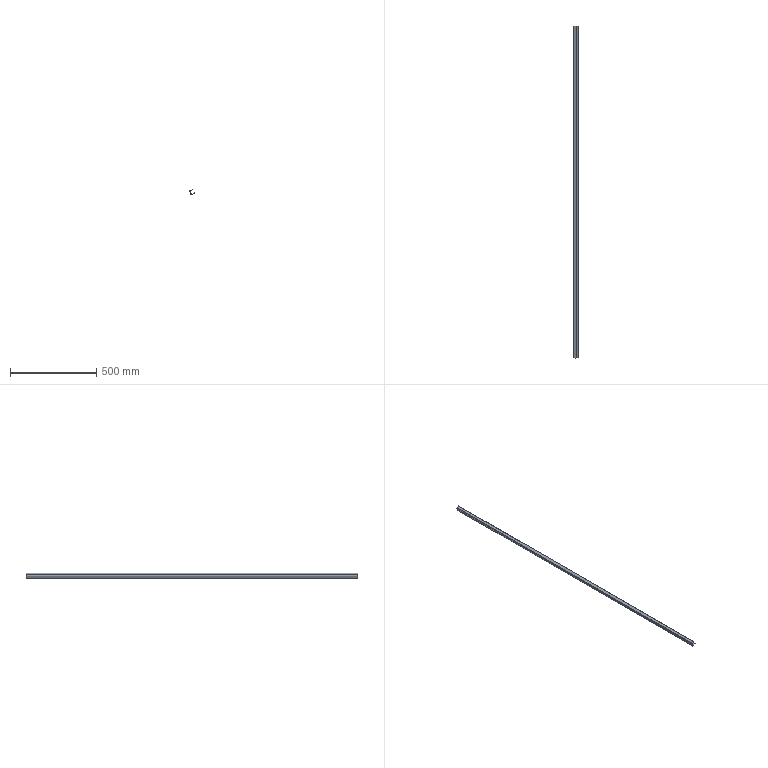Component | SolidWorks | FrontDoorAssembly-1_DoorLeftAndRightReinforcementBar-2 | 1 solid | 22 faces | box 27.81 x 1920 x 29.64 mm | volume 219407 mm3 | plane 18 | cylinder 4 | commonest cylinder face diameters 11 x2 7 x2 | material Malleable Cast Iron
STEP:
#1=COLOUR_RGB('',0.7922,0.8196,0.9333);
#2=FILL_AREA_STYLE_COLOUR('',#1);
#3=FILL_AREA_STYLE('',(#2));
#4=SURFACE_STYLE_FILL_AREA(#3);
#5=SURFACE_SIDE_STYLE('',(#4));
#6=SURFACE_STYLE_USAGE(.BOTH.,#5);
#7=PRESENTATION_STYLE_ASSIGNMENT((#6));
#8=CARTESIAN_POINT('',(-2.645,74.27,40.544));
#9=VERTEX_POINT('',#8);
#10=CARTESIAN_POINT('',(-2.577,74.27,40.583));
#11=VERTEX_POINT('',#10);
#12=CARTESIAN_POINT('',(-2.645,74.27,40.544));
#13=DIRECTION('',(0.866,0.,0.5));
#14=VECTOR('',#13,39.37);
#15=LINE('',#12,#14);
#16=EDGE_CURVE('',#9,#11,#15,.T.);
#17=ORIENTED_EDGE('',*,*,#16,.F.);
#18=CARTESIAN_POINT('',(-2.566,74.27,40.84));
#19=VERTEX_POINT('',#18);
#20=CARTESIAN_POINT('',(-2.458,74.27,40.652));
#21=DIRECTION('',(0.,-1.,-0.));
#22=DIRECTION('',(0.866,0.,0.5));
#23=AXIS2_PLACEMENT_3D('',#20,#21,#22);
#24=CIRCLE('',#23,0.2165);
#25=EDGE_CURVE('',#19,#9,#24,.T.);
#26=ORIENTED_EDGE('',*,*,#25,.F.);
#27=CARTESIAN_POINT('',(-2.527,74.27,40.771));
#28=VERTEX_POINT('',#27);
#29=CARTESIAN_POINT('',(-2.527,74.27,40.771));
#30=DIRECTION('',(-0.5,-0.,0.866));
#31=VECTOR('',#30,39.37);
#32=LINE('',#29,#31);
#33=EDGE_CURVE('',#28,#19,#32,.T.);
#34=ORIENTED_EDGE('',*,*,#33,.F.);
#35=CARTESIAN_POINT('',(-2.458,74.27,40.652));
#36=DIRECTION('',(0.,-1.,-0.));
#37=DIRECTION('',(0.5,0.,-0.866));
#38=AXIS2_PLACEMENT_3D('',#35,#36,#37);
#39=CIRCLE('',#38,0.1378);
#40=EDGE_CURVE('',#28,#11,#39,.T.);
#41=ORIENTED_EDGE('',*,*,#40,.T.);
#42=EDGE_LOOP('',(#17,#26,#34,#41));
#43=FACE_OUTER_BOUND('',#42,.T.);
#44=CARTESIAN_POINT('',(-2.645,74.27,40.544));
#45=DIRECTION('',(-0.,1.,0.));
#46=DIRECTION('',(0.866,0.,0.5));
#47=AXIS2_PLACEMENT_3D('',#44,#45,#46);
#48=PLANE('',#47);
#49=ADVANCED_FACE('',(#43),#48,.T.);
#50=CARTESIAN_POINT('',(-2.37,74.27,40.067));
#51=VERTEX_POINT('',#50);
#52=CARTESIAN_POINT('',(-2.754,74.27,40.731));
#53=DIRECTION('',(0.5,0.,-0.866));
#54=VECTOR('',#53,39.37);
#55=LINE('',#52,#54);
#56=EDGE_CURVE('',#9,#51,#55,.T.);
#57=ORIENTED_EDGE('',*,*,#56,.F.);
#58=ORIENTED_EDGE('',*,*,#16,.T.);
#59=CARTESIAN_POINT('',(-2.302,74.27,40.106));
#60=VERTEX_POINT('',#59);
#61=CARTESIAN_POINT('',(-2.686,74.27,40.771));
#62=DIRECTION('',(0.5,0.,-0.866));
#63=VECTOR('',#62,39.37);
#64=LINE('',#61,#63);
#65=EDGE_CURVE('',#11,#60,#64,.T.);
#66=ORIENTED_EDGE('',*,*,#65,.T.);
#67=CARTESIAN_POINT('',(-2.302,74.27,40.106));
#68=DIRECTION('',(-0.866,-0.,-0.5));
#69=VECTOR('',#68,39.37);
#70=LINE('',#67,#69);
#71=EDGE_CURVE('',#60,#51,#70,.T.);
#72=ORIENTED_EDGE('',*,*,#71,.T.);
#73=EDGE_LOOP('',(#57,#58,#66,#72));
#74=FACE_OUTER_BOUND('',#73,.T.);
#75=CARTESIAN_POINT('',(-2.527,74.27,40.771));
#76=DIRECTION('',(-0.,1.,0.));
#77=DIRECTION('',(0.866,0.,0.5));
#78=AXIS2_PLACEMENT_3D('',#75,#76,#77);
#79=PLANE('',#78);
#80=ADVANCED_FACE('',(#74),#79,.T.);
#81=CARTESIAN_POINT('',(-2.566,-1.32,40.84));
#82=VERTEX_POINT('',#81);
#83=CARTESIAN_POINT('',(-2.527,-1.32,40.771));
#84=VERTEX_POINT('',#83);
#85=CARTESIAN_POINT('',(-2.566,-1.32,40.84));
#86=DIRECTION('',(0.5,0.,-0.866));
#87=VECTOR('',#86,39.37);
#88=LINE('',#85,#87);
#89=EDGE_CURVE('',#82,#84,#88,.T.);
#90=ORIENTED_EDGE('',*,*,#89,.F.);
#91=CARTESIAN_POINT('',(-2.645,-1.32,40.544));
#92=VERTEX_POINT('',#91);
#93=CARTESIAN_POINT('',(-2.458,-1.32,40.652));
#94=DIRECTION('',(0.,-1.,-0.));
#95=DIRECTION('',(0.866,0.,0.5));
#96=AXIS2_PLACEMENT_3D('',#93,#94,#95);
#97=CIRCLE('',#96,0.2165);
#98=EDGE_CURVE('',#82,#92,#97,.T.);
#99=ORIENTED_EDGE('',*,*,#98,.T.);
#100=CARTESIAN_POINT('',(-2.577,-1.32,40.583));
#101=VERTEX_POINT('',#100);
#102=CARTESIAN_POINT('',(-2.577,-1.32,40.583));
#103=DIRECTION('',(-0.866,-0.,-0.5));
#104=VECTOR('',#103,39.37);
#105=LINE('',#102,#104);
#106=EDGE_CURVE('',#101,#92,#105,.T.);
#107=ORIENTED_EDGE('',*,*,#106,.F.);
#108=CARTESIAN_POINT('',(-2.458,-1.32,40.652));
#109=DIRECTION('',(0.,-1.,-0.));
#110=DIRECTION('',(0.5,0.,-0.866));
#111=AXIS2_PLACEMENT_3D('',#108,#109,#110);
#112=CIRCLE('',#111,0.1378);
#113=EDGE_CURVE('',#84,#101,#112,.T.);
#114=ORIENTED_EDGE('',*,*,#113,.F.);
#115=EDGE_LOOP('',(#90,#99,#107,#114));
#116=FACE_OUTER_BOUND('',#115,.T.);
#117=CARTESIAN_POINT('',(-2.566,-1.32,40.84));
#118=DIRECTION('',(0.,-1.,-0.));
#119=DIRECTION('',(-0.866,-0.,-0.5));
#120=AXIS2_PLACEMENT_3D('',#117,#118,#119);
#121=PLANE('',#120);
#122=ADVANCED_FACE('',(#116),#121,.T.);
#123=CARTESIAN_POINT('',(-2.072,-1.32,41.125));
#124=VERTEX_POINT('',#123);
#125=CARTESIAN_POINT('',(-2.072,-1.32,41.125));
#126=DIRECTION('',(-0.866,-0.,-0.5));
#127=VECTOR('',#126,39.37);
#128=LINE('',#125,#127);
#129=EDGE_CURVE('',#124,#82,#128,.T.);
#130=ORIENTED_EDGE('',*,*,#129,.T.);
#131=ORIENTED_EDGE('',*,*,#89,.T.);
#132=CARTESIAN_POINT('',(-2.032,-1.32,41.057));
#133=VERTEX_POINT('',#132);
#134=CARTESIAN_POINT('',(-2.032,-1.32,41.057));
#135=DIRECTION('',(-0.866,-0.,-0.5));
#136=VECTOR('',#135,39.37);
#137=LINE('',#134,#136);
#138=EDGE_CURVE('',#133,#84,#137,.T.);
#139=ORIENTED_EDGE('',*,*,#138,.F.);
#140=CARTESIAN_POINT('',(-2.032,-1.32,41.057));
#141=DIRECTION('',(-0.5,-0.,0.866));
#142=VECTOR('',#141,39.37);
#143=LINE('',#140,#142);
#144=EDGE_CURVE('',#133,#124,#143,.T.);
#145=ORIENTED_EDGE('',*,*,#144,.T.);
#146=EDGE_LOOP('',(#130,#131,#139,#145));
#147=FACE_OUTER_BOUND('',#146,.T.);
#148=CARTESIAN_POINT('',(-2.577,-1.32,40.583));
#149=DIRECTION('',(0.,-1.,-0.));
#150=DIRECTION('',(-0.866,-0.,-0.5));
#151=AXIS2_PLACEMENT_3D('',#148,#149,#150);
#152=PLANE('',#151);
#153=ADVANCED_FACE('',(#147),#152,.T.);
#154=CARTESIAN_POINT('',(-2.074,74.27,39.987));
#155=VERTEX_POINT('',#154);
#156=CARTESIAN_POINT('',(-2.113,74.27,40.055));
#157=VERTEX_POINT('',#156);
#158=CARTESIAN_POINT('',(-2.074,74.27,39.987));
#159=DIRECTION('',(-0.5,-0.,0.866));
#160=VECTOR('',#159,39.37);
#161=LINE('',#158,#160);
#162=EDGE_CURVE('',#155,#157,#161,.T.);
#163=ORIENTED_EDGE('',*,*,#162,.F.);
#164=CARTESIAN_POINT('',(-2.182,74.27,40.175));
#165=DIRECTION('',(0.,-1.,-0.));
#166=DIRECTION('',(0.866,0.,0.5));
#167=AXIS2_PLACEMENT_3D('',#164,#165,#166);
#168=CIRCLE('',#167,0.2165);
#169=EDGE_CURVE('',#51,#155,#168,.T.);
#170=ORIENTED_EDGE('',*,*,#169,.F.);
#171=ORIENTED_EDGE('',*,*,#71,.F.);
#172=CARTESIAN_POINT('',(-2.182,74.27,40.175));
#173=DIRECTION('',(0.,-1.,-0.));
#174=DIRECTION('',(0.5,0.,-0.866));
#175=AXIS2_PLACEMENT_3D('',#172,#173,#174);
#176=CIRCLE('',#175,0.1378);
#177=EDGE_CURVE('',#60,#157,#176,.T.);
#178=ORIENTED_EDGE('',*,*,#177,.T.);
#179=EDGE_LOOP('',(#163,#170,#171,#178));
#180=FACE_OUTER_BOUND('',#179,.T.);
#181=CARTESIAN_POINT('',(-2.074,74.27,39.987));
#182=DIRECTION('',(-0.,1.,0.));
#183=DIRECTION('',(0.866,0.,0.5));
#184=AXIS2_PLACEMENT_3D('',#181,#182,#183);
#185=PLANE('',#184);
#186=ADVANCED_FACE('',(#180),#185,.T.);
#187=CARTESIAN_POINT('',(-1.58,74.27,40.273));
#188=VERTEX_POINT('',#187);
#189=CARTESIAN_POINT('',(-2.262,74.27,39.879));
#190=DIRECTION('',(0.866,0.,0.5));
#191=VECTOR('',#190,39.37);
#192=LINE('',#189,#191);
#193=EDGE_CURVE('',#155,#188,#192,.T.);
#194=ORIENTED_EDGE('',*,*,#193,.F.);
#195=ORIENTED_EDGE('',*,*,#162,.T.);
#196=CARTESIAN_POINT('',(-1.619,74.27,40.341));
#197=VERTEX_POINT('',#196);
#198=CARTESIAN_POINT('',(-2.301,74.27,39.947));
#199=DIRECTION('',(0.866,0.,0.5));
#200=VECTOR('',#199,39.37);
#201=LINE('',#198,#200);
#202=EDGE_CURVE('',#157,#197,#201,.T.);
#203=ORIENTED_EDGE('',*,*,#202,.T.);
#204=CARTESIAN_POINT('',(-1.58,74.27,40.273));
#205=DIRECTION('',(-0.5,-0.,0.866));
#206=VECTOR('',#205,39.37);
#207=LINE('',#204,#206);
#208=EDGE_CURVE('',#188,#197,#207,.T.);
#209=ORIENTED_EDGE('',*,*,#208,.F.);
#210=EDGE_LOOP('',(#194,#195,#203,#209));
#211=FACE_OUTER_BOUND('',#210,.T.);
#212=CARTESIAN_POINT('',(-2.302,74.27,40.106));
#213=DIRECTION('',(-0.,1.,0.));
#214=DIRECTION('',(0.866,0.,0.5));
#215=AXIS2_PLACEMENT_3D('',#212,#213,#214);
#216=PLANE('',#215);
#217=ADVANCED_FACE('',(#211),#216,.T.);
#218=CARTESIAN_POINT('',(-2.37,-1.32,40.067));
#219=VERTEX_POINT('',#218);
#220=CARTESIAN_POINT('',(-2.302,-1.32,40.106));
#221=VERTEX_POINT('',#220);
#222=CARTESIAN_POINT('',(-2.37,-1.32,40.067));
#223=DIRECTION('',(0.866,0.,0.5));
#224=VECTOR('',#223,39.37);
#225=LINE('',#222,#224);
#226=EDGE_CURVE('',#219,#221,#225,.T.);
#227=ORIENTED_EDGE('',*,*,#226,.F.);
#228=CARTESIAN_POINT('',(-2.074,-1.32,39.987));
#229=VERTEX_POINT('',#228);
#230=CARTESIAN_POINT('',(-2.182,-1.32,40.175));
#231=DIRECTION('',(0.,-1.,-0.));
#232=DIRECTION('',(0.866,0.,0.5));
#233=AXIS2_PLACEMENT_3D('',#230,#231,#232);
#234=CIRCLE('',#233,0.2165);
#235=EDGE_CURVE('',#219,#229,#234,.T.);
#236=ORIENTED_EDGE('',*,*,#235,.T.);
#237=CARTESIAN_POINT('',(-2.113,-1.32,40.055));
#238=VERTEX_POINT('',#237);
#239=CARTESIAN_POINT('',(-2.113,-1.32,40.055));
#240=DIRECTION('',(0.5,0.,-0.866));
#241=VECTOR('',#240,39.37);
#242=LINE('',#239,#241);
#243=EDGE_CURVE('',#238,#229,#242,.T.);
#244=ORIENTED_EDGE('',*,*,#243,.F.);
#245=CARTESIAN_POINT('',(-2.182,-1.32,40.175));
#246=DIRECTION('',(0.,-1.,-0.));
#247=DIRECTION('',(0.5,0.,-0.866));
#248=AXIS2_PLACEMENT_3D('',#245,#246,#247);
#249=CIRCLE('',#248,0.1378);
#250=EDGE_CURVE('',#221,#238,#249,.T.);
#251=ORIENTED_EDGE('',*,*,#250,.F.);
#252=EDGE_LOOP('',(#227,#236,#244,#251));
#253=FACE_OUTER_BOUND('',#252,.T.);
#254=CARTESIAN_POINT('',(-2.37,-1.32,40.067));
#255=DIRECTION('',(0.,-1.,-0.));
#256=DIRECTION('',(-0.866,-0.,-0.5));
#257=AXIS2_PLACEMENT_3D('',#254,#255,#256);
#258=PLANE('',#257);
#259=ADVANCED_FACE('',(#253),#258,.T.);
#260=CARTESIAN_POINT('',(-2.754,-1.32,40.731));
#261=DIRECTION('',(0.5,0.,-0.866));
#262=VECTOR('',#261,39.37);
#263=LINE('',#260,#262);
#264=EDGE_CURVE('',#92,#219,#263,.T.);
#265=ORIENTED_EDGE('',*,*,#264,.T.);
#266=ORIENTED_EDGE('',*,*,#226,.T.);
#267=CARTESIAN_POINT('',(-2.686,-1.32,40.771));
#268=DIRECTION('',(0.5,0.,-0.866));
#269=VECTOR('',#268,39.37);
#270=LINE('',#267,#269);
#271=EDGE_CURVE('',#101,#221,#270,.T.);
#272=ORIENTED_EDGE('',*,*,#271,.F.);
#273=ORIENTED_EDGE('',*,*,#106,.T.);
#274=EDGE_LOOP('',(#265,#266,#272,#273));
#275=FACE_OUTER_BOUND('',#274,.T.);
#276=CARTESIAN_POINT('',(-2.113,-1.32,40.055));
#277=DIRECTION('',(0.,-1.,-0.));
#278=DIRECTION('',(-0.866,-0.,-0.5));
#279=AXIS2_PLACEMENT_3D('',#276,#277,#278);
#280=PLANE('',#279);
#281=ADVANCED_FACE('',(#275),#280,.T.);
#282=CARTESIAN_POINT('',(-1.619,-1.32,40.341));
#283=VERTEX_POINT('',#282);
#284=CARTESIAN_POINT('',(-2.301,-1.32,39.947));
#285=DIRECTION('',(0.866,0.,0.5));
#286=VECTOR('',#285,39.37);
#287=LINE('',#284,#286);
#288=EDGE_CURVE('',#238,#283,#287,.T.);
#289=ORIENTED_EDGE('',*,*,#288,.T.);
#290=CARTESIAN_POINT('',(-1.619,74.27,40.341));
#291=DIRECTION('',(0.,-1.,-0.));
#292=VECTOR('',#291,39.37);
#293=LINE('',#290,#292);
#294=EDGE_CURVE('',#197,#283,#293,.T.);
#295=ORIENTED_EDGE('',*,*,#294,.F.);
#296=ORIENTED_EDGE('',*,*,#202,.F.);
#297=CARTESIAN_POINT('',(-2.113,74.27,40.055));
#298=DIRECTION('',(0.,-1.,-0.));
#299=VECTOR('',#298,39.37);
#300=LINE('',#297,#299);
#301=EDGE_CURVE('',#157,#238,#300,.T.);
#302=ORIENTED_EDGE('',*,*,#301,.T.);
#303=EDGE_LOOP('',(#289,#295,#296,#302));
#304=FACE_OUTER_BOUND('',#303,.T.);
#305=CARTESIAN_POINT('',(-2.301,74.27,39.947));
#306=DIRECTION('',(0.5,0.,-0.866));
#307=DIRECTION('',(-0.866,-0.,-0.5));
#308=AXIS2_PLACEMENT_3D('',#305,#306,#307);
#309=PLANE('',#308);
#310=ADVANCED_FACE('',(#304),#309,.F.);
#311=CARTESIAN_POINT('',(-1.58,-1.32,40.273));
#312=VERTEX_POINT('',#311);
#313=CARTESIAN_POINT('',(-1.58,-1.32,40.273));
#314=DIRECTION('',(-0.5,-0.,0.866));
#315=VECTOR('',#314,39.37);
#316=LINE('',#313,#315);
#317=EDGE_CURVE('',#312,#283,#316,.T.);
#318=ORIENTED_EDGE('',*,*,#317,.F.);
#319=CARTESIAN_POINT('',(-1.58,74.27,40.273));
#320=DIRECTION('',(0.,-1.,-0.));
#321=VECTOR('',#320,39.37);
#322=LINE('',#319,#321);
#323=EDGE_CURVE('',#188,#312,#322,.T.);
#324=ORIENTED_EDGE('',*,*,#323,.F.);
#325=ORIENTED_EDGE('',*,*,#208,.T.);
#326=ORIENTED_EDGE('',*,*,#294,.T.);
#327=EDGE_LOOP('',(#318,#324,#325,#326));
#328=FACE_OUTER_BOUND('',#327,.T.);
#329=CARTESIAN_POINT('',(-1.58,74.27,40.273));
#330=DIRECTION('',(0.866,0.,0.5));
#331=DIRECTION('',(0.5,0.,-0.866));
#332=AXIS2_PLACEMENT_3D('',#329,#330,#331);
#333=PLANE('',#332);
#334=ADVANCED_FACE('',(#328),#333,.T.);
#335=CARTESIAN_POINT('',(-2.262,-1.32,39.879));
#336=DIRECTION('',(0.866,0.,0.5));
#337=VECTOR('',#336,39.37);
#338=LINE('',#335,#337);
#339=EDGE_CURVE('',#229,#312,#338,.T.);
#340=ORIENTED_EDGE('',*,*,#339,.F.);
#341=CARTESIAN_POINT('',(-2.074,74.27,39.987));
#342=DIRECTION('',(0.,-1.,-0.));
#343=VECTOR('',#342,39.37);
#344=LINE('',#341,#343);
#345=EDGE_CURVE('',#155,#229,#344,.T.);
#346=ORIENTED_EDGE('',*,*,#345,.F.);
#347=ORIENTED_EDGE('',*,*,#193,.T.);
#348=ORIENTED_EDGE('',*,*,#323,.T.);
#349=EDGE_LOOP('',(#340,#346,#347,#348));
#350=FACE_OUTER_BOUND('',#349,.T.);
#351=CARTESIAN_POINT('',(-2.262,74.27,39.879));
#352=DIRECTION('',(0.5,0.,-0.866));
#353=DIRECTION('',(-0.866,-0.,-0.5));
#354=AXIS2_PLACEMENT_3D('',#351,#352,#353);
#355=PLANE('',#354);
#356=ADVANCED_FACE('',(#350),#355,.T.);
#357=ORIENTED_EDGE('',*,*,#235,.F.);
#358=CARTESIAN_POINT('',(-2.37,74.27,40.067));
#359=DIRECTION('',(0.,-1.,-0.));
#360=VECTOR('',#359,39.37);
#361=LINE('',#358,#360);
#362=EDGE_CURVE('',#51,#219,#361,.T.);
#363=ORIENTED_EDGE('',*,*,#362,.F.);
#364=ORIENTED_EDGE('',*,*,#169,.T.);
#365=ORIENTED_EDGE('',*,*,#345,.T.);
#366=EDGE_LOOP('',(#357,#363,#364,#365));
#367=FACE_OUTER_BOUND('',#366,.T.);
#368=CARTESIAN_POINT('',(-2.182,74.27,40.175));
#369=DIRECTION('',(0.,-1.,-0.));
#370=DIRECTION('',(-0.866,0.,-0.5));
#371=AXIS2_PLACEMENT_3D('',#368,#369,#370);
#372=CYLINDRICAL_SURFACE('',#371,0.2165);
#373=ADVANCED_FACE('',(#367),#372,.T.);
#374=ORIENTED_EDGE('',*,*,#264,.F.);
#375=CARTESIAN_POINT('',(-2.645,74.27,40.544));
#376=DIRECTION('',(0.,-1.,-0.));
#377=VECTOR('',#376,39.37);
#378=LINE('',#375,#377);
#379=EDGE_CURVE('',#9,#92,#378,.T.);
#380=ORIENTED_EDGE('',*,*,#379,.F.);
#381=ORIENTED_EDGE('',*,*,#56,.T.);
#382=ORIENTED_EDGE('',*,*,#362,.T.);
#383=EDGE_LOOP('',(#374,#380,#381,#382));
#384=FACE_OUTER_BOUND('',#383,.T.);
#385=CARTESIAN_POINT('',(-2.754,74.27,40.731));
#386=DIRECTION('',(-0.866,-0.,-0.5));
#387=DIRECTION('',(-0.5,-0.,0.866));
#388=AXIS2_PLACEMENT_3D('',#385,#386,#387);
#389=PLANE('',#388);
#390=ADVANCED_FACE('',(#384),#389,.T.);
#391=ORIENTED_EDGE('',*,*,#98,.F.);
#392=CARTESIAN_POINT('',(-2.566,74.27,40.84));
#393=DIRECTION('',(0.,-1.,-0.));
#394=VECTOR('',#393,39.37);
#395=LINE('',#392,#394);
#396=EDGE_CURVE('',#19,#82,#395,.T.);
#397=ORIENTED_EDGE('',*,*,#396,.F.);
#398=ORIENTED_EDGE('',*,*,#25,.T.);
#399=ORIENTED_EDGE('',*,*,#379,.T.);
#400=EDGE_LOOP('',(#391,#397,#398,#399));
#401=FACE_OUTER_BOUND('',#400,.T.);
#402=CARTESIAN_POINT('',(-2.458,74.27,40.652));
#403=DIRECTION('',(0.,-1.,-0.));
#404=DIRECTION('',(-0.866,0.,-0.5));
#405=AXIS2_PLACEMENT_3D('',#402,#403,#404);
#406=CYLINDRICAL_SURFACE('',#405,0.2165);
#407=ADVANCED_FACE('',(#401),#406,.T.);
#408=ORIENTED_EDGE('',*,*,#129,.F.);
#409=CARTESIAN_POINT('',(-2.072,74.27,41.125));
#410=VERTEX_POINT('',#409);
#411=CARTESIAN_POINT('',(-2.072,74.27,41.125));
#412=DIRECTION('',(0.,-1.,-0.));
#413=VECTOR('',#412,39.37);
#414=LINE('',#411,#413);
#415=EDGE_CURVE('',#410,#124,#414,.T.);
#416=ORIENTED_EDGE('',*,*,#415,.F.);
#417=CARTESIAN_POINT('',(-2.072,74.27,41.125));
#418=DIRECTION('',(-0.866,-0.,-0.5));
#419=VECTOR('',#418,39.37);
#420=LINE('',#417,#419);
#421=EDGE_CURVE('',#410,#19,#420,.T.);
#422=ORIENTED_EDGE('',*,*,#421,.T.);
#423=ORIENTED_EDGE('',*,*,#396,.T.);
#424=EDGE_LOOP('',(#408,#416,#422,#423));
#425=FACE_OUTER_BOUND('',#424,.T.);
#426=CARTESIAN_POINT('',(-2.072,74.27,41.125));
#427=DIRECTION('',(-0.5,-0.,0.866));
#428=DIRECTION('',(0.866,0.,0.5));
#429=AXIS2_PLACEMENT_3D('',#426,#427,#428);
#430=PLANE('',#429);
#431=ADVANCED_FACE('',(#425),#430,.T.);
#432=ORIENTED_EDGE('',*,*,#144,.F.);
#433=CARTESIAN_POINT('',(-2.032,74.27,41.057));
#434=VERTEX_POINT('',#433);
#435=CARTESIAN_POINT('',(-2.032,74.27,41.057));
#436=DIRECTION('',(0.,-1.,-0.));
#437=VECTOR('',#436,39.37);
#438=LINE('',#435,#437);
#439=EDGE_CURVE('',#434,#133,#438,.T.);
#440=ORIENTED_EDGE('',*,*,#439,.F.);
#441=CARTESIAN_POINT('',(-2.032,74.27,41.057));
#442=DIRECTION('',(-0.5,-0.,0.866));
#443=VECTOR('',#442,39.37);
#444=LINE('',#441,#443);
#445=EDGE_CURVE('',#434,#410,#444,.T.);
#446=ORIENTED_EDGE('',*,*,#445,.T.);
#447=ORIENTED_EDGE('',*,*,#415,.T.);
#448=EDGE_LOOP('',(#432,#440,#446,#447));
#449=FACE_OUTER_BOUND('',#448,.T.);
#450=CARTESIAN_POINT('',(-2.032,74.27,41.057));
#451=DIRECTION('',(0.866,0.,0.5));
#452=DIRECTION('',(0.5,0.,-0.866));
#453=AXIS2_PLACEMENT_3D('',#450,#451,#452);
#454=PLANE('',#453);
#455=ADVANCED_FACE('',(#449),#454,.T.);
#456=ORIENTED_EDGE('',*,*,#138,.T.);
#457=CARTESIAN_POINT('',(-2.527,74.27,40.771));
#458=DIRECTION('',(0.,-1.,-0.));
#459=VECTOR('',#458,39.37);
#460=LINE('',#457,#459);
#461=EDGE_CURVE('',#28,#84,#460,.T.);
#462=ORIENTED_EDGE('',*,*,#461,.F.);
#463=CARTESIAN_POINT('',(-2.032,74.27,41.057));
#464=DIRECTION('',(-0.866,-0.,-0.5));
#465=VECTOR('',#464,39.37);
#466=LINE('',#463,#465);
#467=EDGE_CURVE('',#434,#28,#466,.T.);
#468=ORIENTED_EDGE('',*,*,#467,.F.);
#469=ORIENTED_EDGE('',*,*,#439,.T.);
#470=EDGE_LOOP('',(#456,#462,#468,#469));
#471=FACE_OUTER_BOUND('',#470,.T.);
#472=CARTESIAN_POINT('',(-2.032,74.27,41.057));
#473=DIRECTION('',(-0.5,-0.,0.866));
#474=DIRECTION('',(0.866,0.,0.5));
#475=AXIS2_PLACEMENT_3D('',#472,#473,#474);
#476=PLANE('',#475);
#477=ADVANCED_FACE('',(#471),#476,.F.);
#478=ORIENTED_EDGE('',*,*,#113,.T.);
#479=CARTESIAN_POINT('',(-2.577,74.27,40.583));
#480=DIRECTION('',(0.,-1.,-0.));
#481=VECTOR('',#480,39.37);
#482=LINE('',#479,#481);
#483=EDGE_CURVE('',#11,#101,#482,.T.);
#484=ORIENTED_EDGE('',*,*,#483,.F.);
#485=ORIENTED_EDGE('',*,*,#40,.F.);
#486=ORIENTED_EDGE('',*,*,#461,.T.);
#487=EDGE_LOOP('',(#478,#484,#485,#486));
#488=FACE_OUTER_BOUND('',#487,.T.);
#489=CARTESIAN_POINT('',(-2.458,74.27,40.652));
#490=DIRECTION('',(0.,-1.,-0.));
#491=DIRECTION('',(-0.866,0.,-0.5));
#492=AXIS2_PLACEMENT_3D('',#489,#490,#491);
#493=CYLINDRICAL_SURFACE('',#492,0.1378);
#494=ADVANCED_FACE('',(#488),#493,.F.);
#495=ORIENTED_EDGE('',*,*,#271,.T.);
#496=CARTESIAN_POINT('',(-2.302,74.27,40.106));
#497=DIRECTION('',(0.,-1.,-0.));
#498=VECTOR('',#497,39.37);
#499=LINE('',#496,#498);
#500=EDGE_CURVE('',#60,#221,#499,.T.);
#501=ORIENTED_EDGE('',*,*,#500,.F.);
#502=ORIENTED_EDGE('',*,*,#65,.F.);
#503=ORIENTED_EDGE('',*,*,#483,.T.);
#504=EDGE_LOOP('',(#495,#501,#502,#503));
#505=FACE_OUTER_BOUND('',#504,.T.);
#506=CARTESIAN_POINT('',(-2.686,74.27,40.771));
#507=DIRECTION('',(-0.866,-0.,-0.5));
#508=DIRECTION('',(-0.5,-0.,0.866));
#509=AXIS2_PLACEMENT_3D('',#506,#507,#508);
#510=PLANE('',#509);
#511=ADVANCED_FACE('',(#505),#510,.F.);
#512=ORIENTED_EDGE('',*,*,#250,.T.);
#513=ORIENTED_EDGE('',*,*,#301,.F.);
#514=ORIENTED_EDGE('',*,*,#177,.F.);
#515=ORIENTED_EDGE('',*,*,#500,.T.);
#516=EDGE_LOOP('',(#512,#513,#514,#515));
#517=FACE_OUTER_BOUND('',#516,.T.);
#518=CARTESIAN_POINT('',(-2.182,74.27,40.175));
#519=DIRECTION('',(0.,-1.,-0.));
#520=DIRECTION('',(-0.866,0.,-0.5));
#521=AXIS2_PLACEMENT_3D('',#518,#519,#520);
#522=CYLINDRICAL_SURFACE('',#521,0.1378);
#523=ADVANCED_FACE('',(#517),#522,.F.);
#524=ORIENTED_EDGE('',*,*,#467,.T.);
#525=ORIENTED_EDGE('',*,*,#33,.T.);
#526=ORIENTED_EDGE('',*,*,#421,.F.);
#527=ORIENTED_EDGE('',*,*,#445,.F.);
#528=EDGE_LOOP('',(#524,#525,#526,#527));
#529=FACE_OUTER_BOUND('',#528,.T.);
#530=CARTESIAN_POINT('',(-2.182,74.27,40.175));
#531=DIRECTION('',(-0.,1.,0.));
#532=DIRECTION('',(0.5,0.,-0.866));
#533=AXIS2_PLACEMENT_3D('',#530,#531,#532);
#534=PLANE('',#533);
#535=ADVANCED_FACE('',(#529),#534,.T.);
#536=ORIENTED_EDGE('',*,*,#288,.F.);
#537=ORIENTED_EDGE('',*,*,#243,.T.);
#538=ORIENTED_EDGE('',*,*,#339,.T.);
#539=ORIENTED_EDGE('',*,*,#317,.T.);
#540=EDGE_LOOP('',(#536,#537,#538,#539));
#541=FACE_OUTER_BOUND('',#540,.T.);
#542=CARTESIAN_POINT('',(-2.182,-1.32,40.175));
#543=DIRECTION('',(-0.,1.,0.));
#544=DIRECTION('',(0.5,0.,-0.866));
#545=AXIS2_PLACEMENT_3D('',#542,#543,#544);
#546=PLANE('',#545);
#547=ADVANCED_FACE('',(#541),#546,.F.);
#548=CLOSED_SHELL('',(#49,#80,#122,#153,#186,#217,#259,#281,#310,#334,#356,#373,#390,#407,#431,#455,#477,#494,#511,#523,#535,#547));
#549=MANIFOLD_SOLID_BREP('',#548);
#550=STYLED_ITEM('',(#7),#549);
#551=PRESENTATION_LAYER_ASSIGNMENT('','',(#550));
#552=CARTESIAN_POINT('',(0.,0.,0.));
#553=DIRECTION('',(0.,0.,1.));
#554=DIRECTION('',(1.,0.,0.));
#555=AXIS2_PLACEMENT_3D('',#552,#553,#554);
#556=(LENGTH_UNIT()NAMED_UNIT(*)SI_UNIT($,.METRE.));
#557=LENGTH_MEASURE_WITH_UNIT(LENGTH_MEASURE(0.0254),#556);
#558=DIMENSIONAL_EXPONENTS(1.,0.,0.,0.,0.,0.,0.);
#559=(CONVERSION_BASED_UNIT('',#557)LENGTH_UNIT()NAMED_UNIT(#558));
#560=UNCERTAINTY_MEASURE_WITH_UNIT(LENGTH_MEASURE(0.00001),#559,'','');
#561=(NAMED_UNIT(*)PLANE_ANGLE_UNIT()SI_UNIT($,.RADIAN.));
#562=(NAMED_UNIT(*)SI_UNIT($,.STERADIAN.)SOLID_ANGLE_UNIT());
#563=(GEOMETRIC_REPRESENTATION_CONTEXT(3)GLOBAL_UNCERTAINTY_ASSIGNED_CONTEXT((#560))GLOBAL_UNIT_ASSIGNED_CONTEXT((#559,#561,#562))REPRESENTATION_CONTEXT('',''));
#564=ADVANCED_BREP_SHAPE_REPRESENTATION('',(#549,#555),#563);
#565=(LENGTH_UNIT()NAMED_UNIT(*)SI_UNIT($,.METRE.));
#566=LENGTH_MEASURE_WITH_UNIT(LENGTH_MEASURE(0.0254),#565);
#567=DIMENSIONAL_EXPONENTS(1.,0.,0.,0.,0.,0.,0.);
#568=(CONVERSION_BASED_UNIT('',#566)LENGTH_UNIT()NAMED_UNIT(#567));
#569=UNCERTAINTY_MEASURE_WITH_UNIT(LENGTH_MEASURE(0.00001),#568,'','');
#570=(NAMED_UNIT(*)PLANE_ANGLE_UNIT()SI_UNIT($,.RADIAN.));
#571=(NAMED_UNIT(*)SI_UNIT($,.STERADIAN.)SOLID_ANGLE_UNIT());
#572=(GEOMETRIC_REPRESENTATION_CONTEXT(3)GLOBAL_UNCERTAINTY_ASSIGNED_CONTEXT((#569))GLOBAL_UNIT_ASSIGNED_CONTEXT((#568,#570,#571))REPRESENTATION_CONTEXT('',''));
#573=MECHANICAL_DESIGN_GEOMETRIC_PRESENTATION_REPRESENTATION('',(#550),#572);